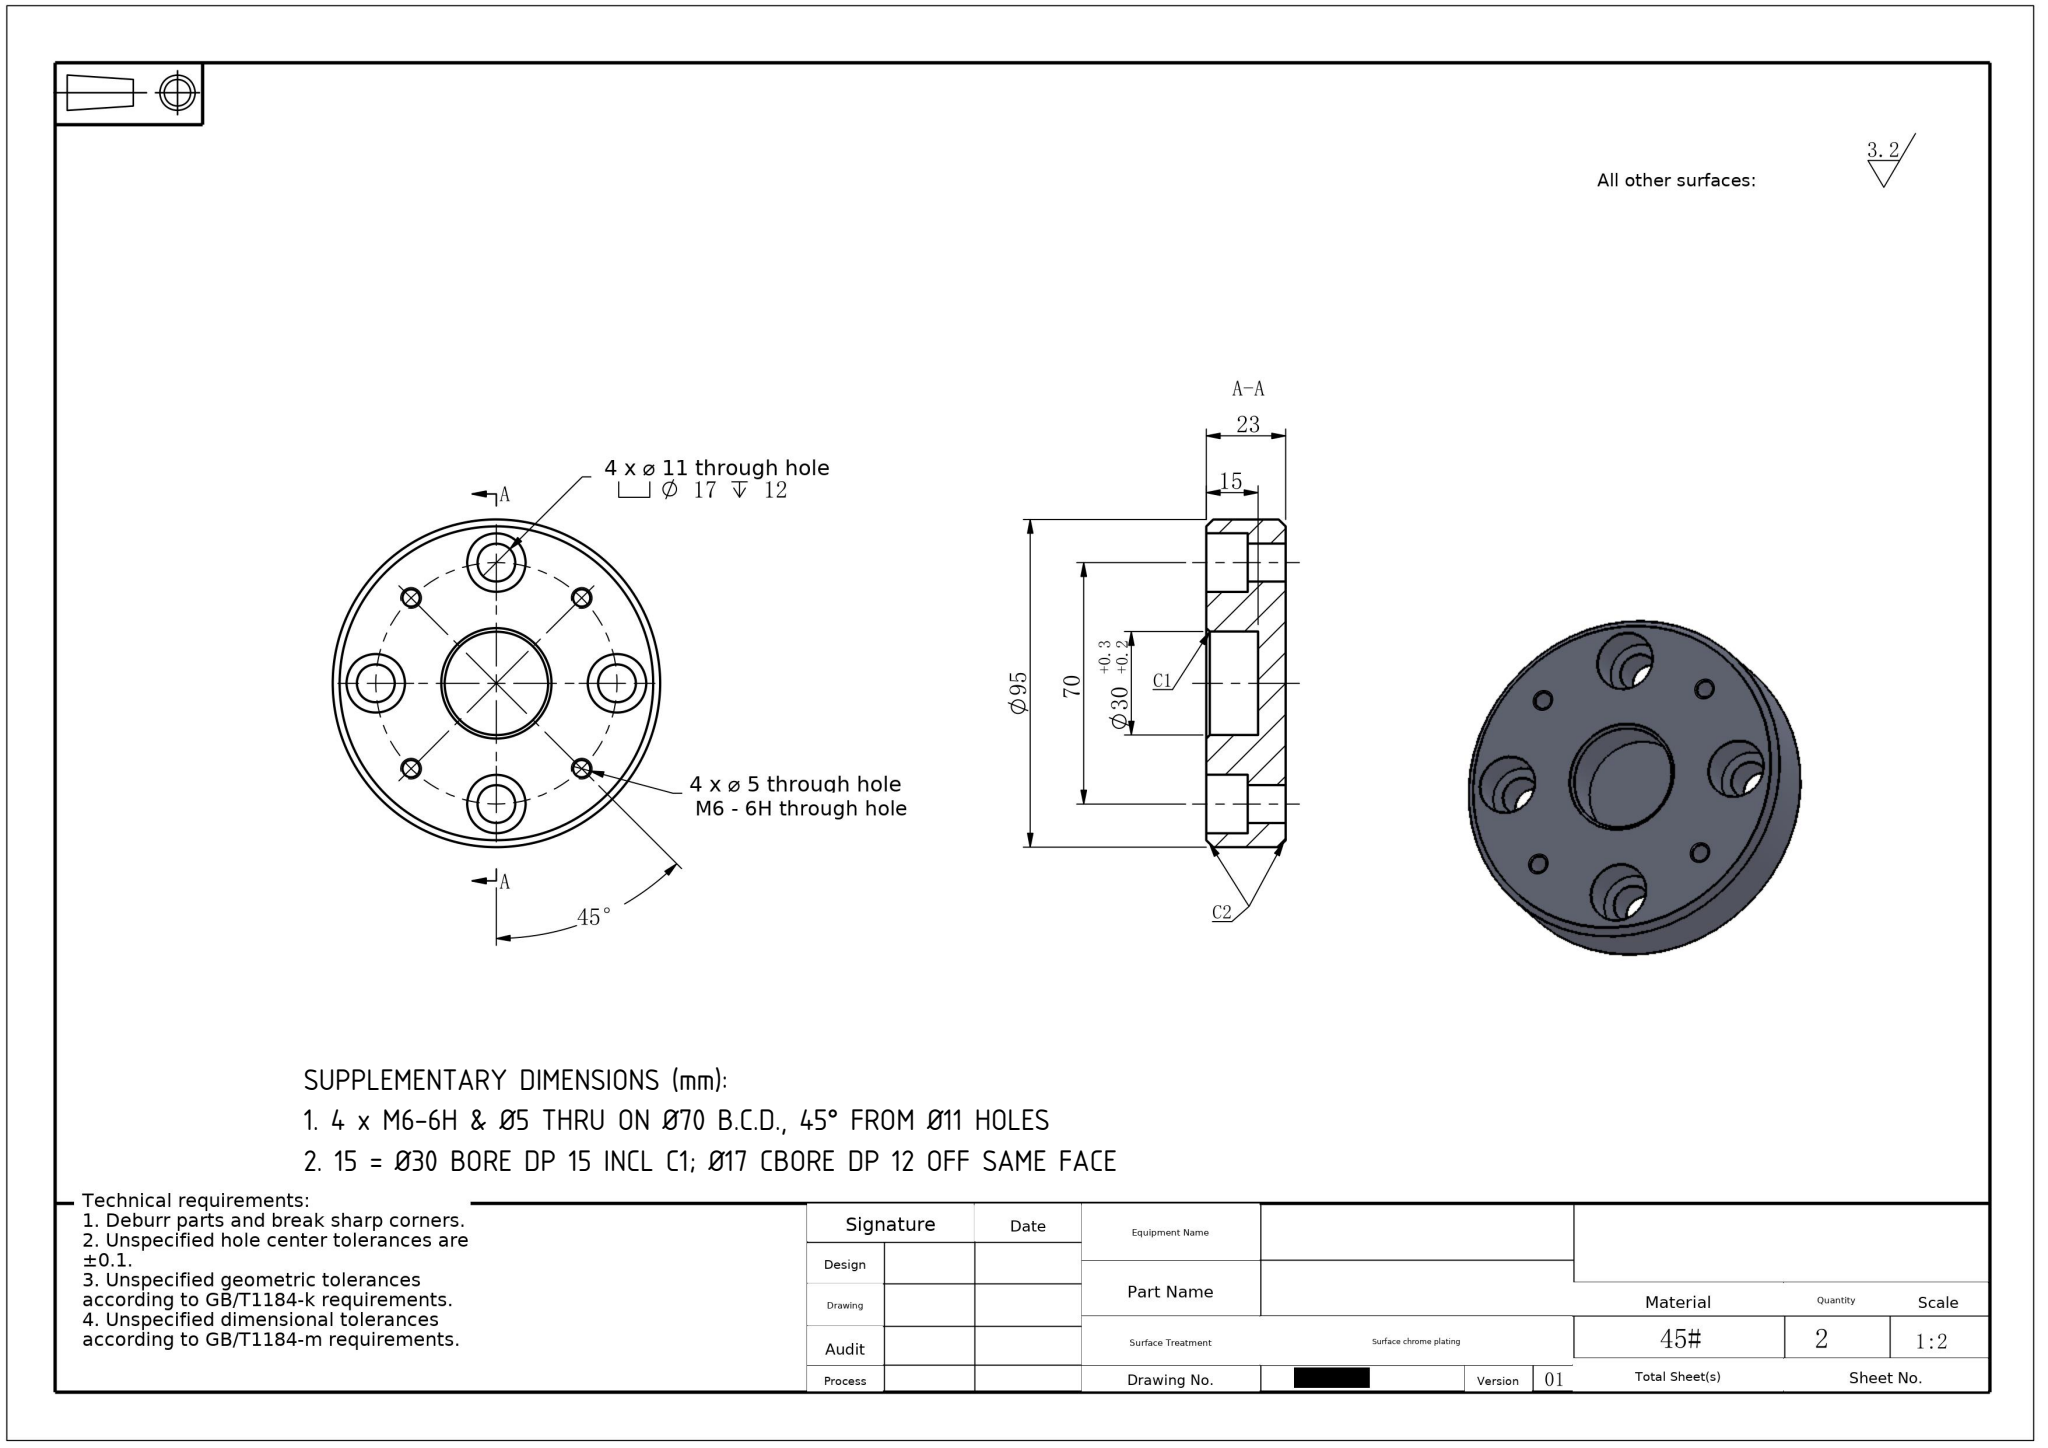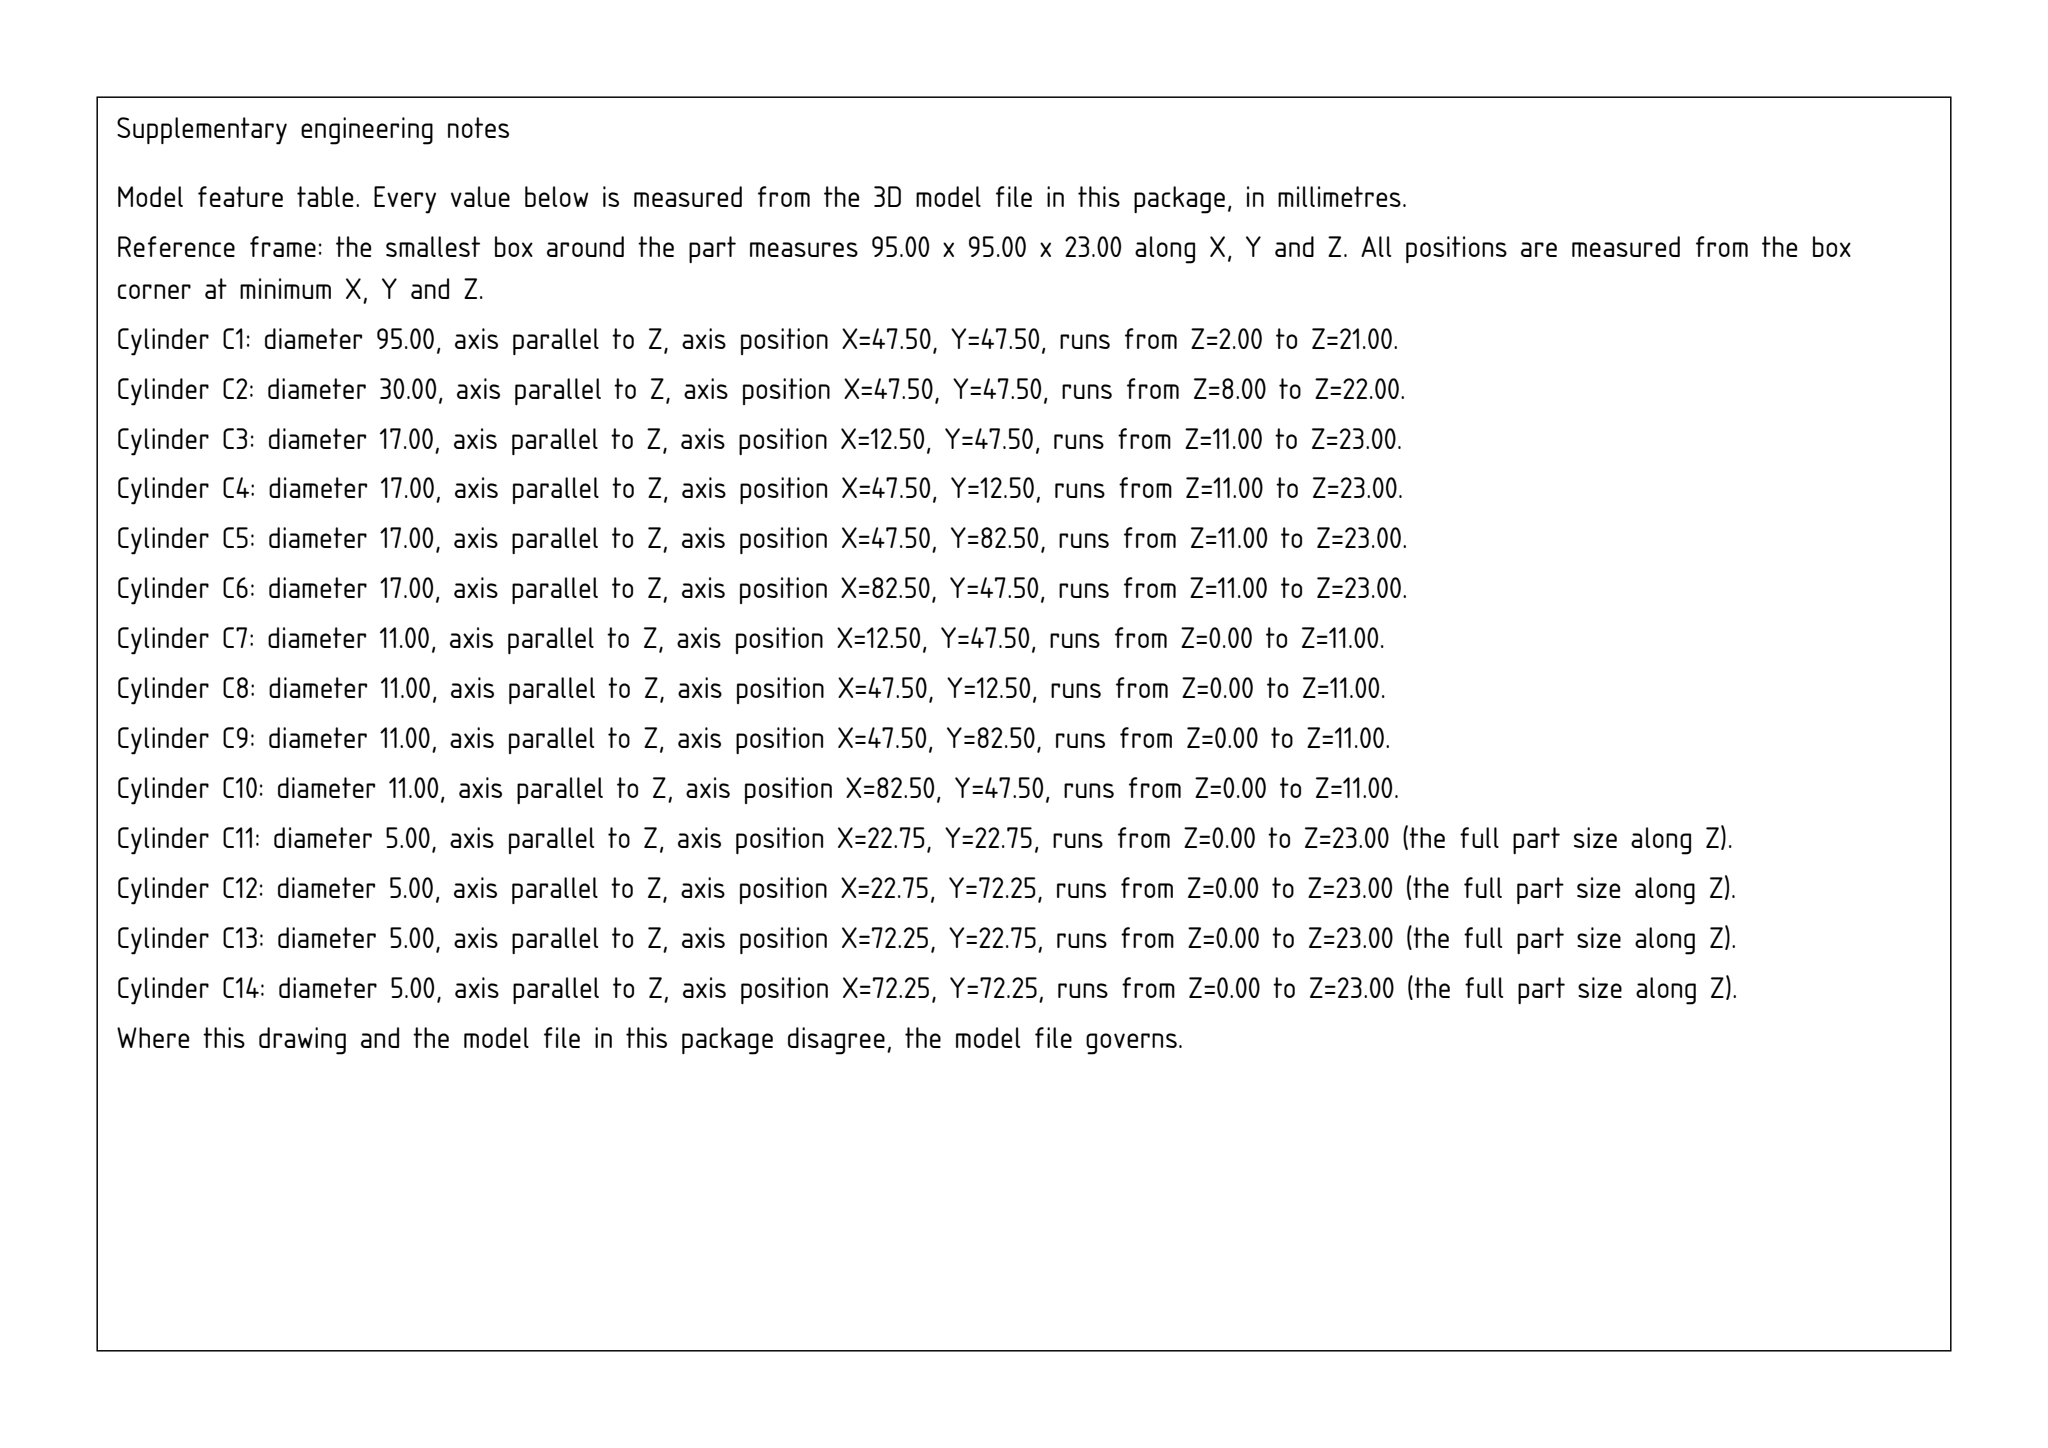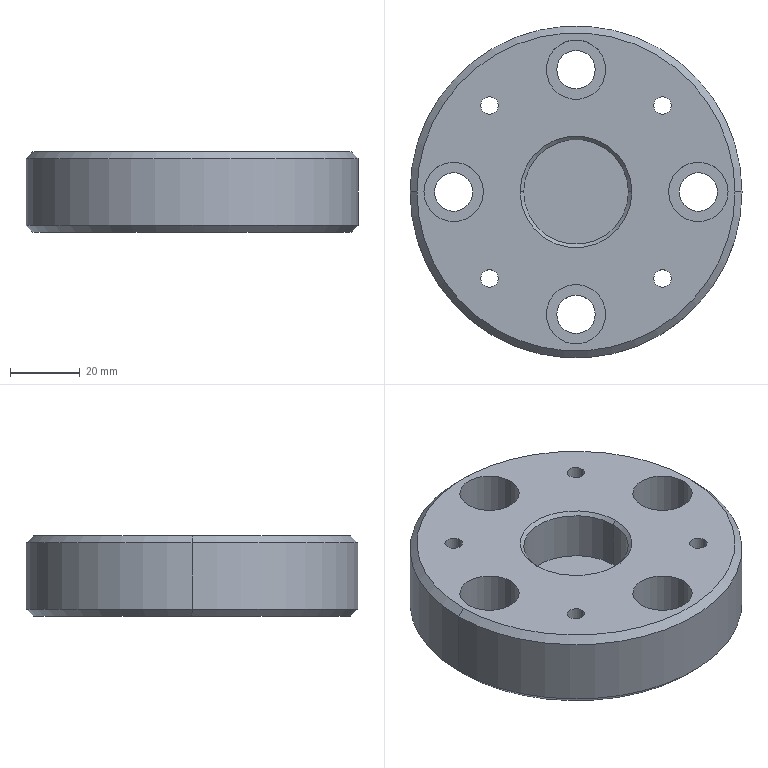Part | SolidWorks | mm | 1 solid | 41 faces | box 95 x 95 x 23 mm | volume 134318 mm3 | cylinder 28 | plane 7 | cone 6 | commonest cylinder face diameters 5 x8 17 x8 11 x8 30 x2 95 x2
build123d program:
from build123d import *

# Parameters (mm, degrees)
SKETCH1_R                                        = 47.5
BOSS_EXTRUDE1_DEPTH                              = 23
SKETCH2_R                                        = 15
CUT_EXTRUDE1_DEPTH                               = 15
CHAMFER1_SIZE                                    = 1
M10_HEX_SOCKET_HEAD_CAP_SCREW_CBORE1_D           = 11
M10_HEX_SOCKET_HEAD_CAP_SCREW_CBORE1_CBORE_D     = 17
M10_HEX_SOCKET_HEAD_CAP_SCREW_CBORE1_CBORE_DEPTH = 12
CIRPATTERN1_COUNT                                = 4
M6_TAPPED_HOLE1_D                                = 5
CIRPATTERN2_COUNT                                = 4
CHAMFER2_SIZE                                    = 2


with BuildPart() as part:
    # Sketch1 → Boss-Extrude1 (new body)
    with BuildSketch(Plane.XY):
        Circle(SKETCH1_R)
    extrude(amount=BOSS_EXTRUDE1_DEPTH)

    # Sketch2 → Cut-Extrude1 (cut)
    with BuildSketch(Plane.XY.offset(23)):
        Circle(SKETCH2_R)
    extrude(amount=-CUT_EXTRUDE1_DEPTH, mode=Mode.SUBTRACT)

    # Chamfer1
    chamfer1_edges = [part.edges().sort_by_distance(p)[0] for p in [
        (-15, 0, 23),
    ]]
    chamfer(chamfer1_edges, length=CHAMFER1_SIZE)

    # M10 Hex Socket Head Cap Screw CBORE1 (through all)
    with Locations(Plane.XY.offset(23)):
        with Locations((0, 35)):
            m10_hex_socket_head_cap_screw_cbore1 = CounterBoreHole(M10_HEX_SOCKET_HEAD_CAP_SCREW_CBORE1_D / 2, M10_HEX_SOCKET_HEAD_CAP_SCREW_CBORE1_CBORE_D / 2, M10_HEX_SOCKET_HEAD_CAP_SCREW_CBORE1_CBORE_DEPTH)

    # CirPattern1: M10 Hex Socket Head Cap Screw CBORE1 ×4 about axis
    cirpattern1_axis = Axis((0, 0, 0), (0, 0, 1))
    for i in range(1, CIRPATTERN1_COUNT):
        add(m10_hex_socket_head_cap_screw_cbore1.rotate(cirpattern1_axis, i * 360 / CIRPATTERN1_COUNT), mode=Mode.SUBTRACT)

    # M6 Tapped Hole1 (through all)
    with Locations(Plane.XY.offset(23)):
        with Locations((-24.749, -24.749)):
            m6_tapped_hole1 = Hole(M6_TAPPED_HOLE1_D / 2)

    # CirPattern2: M6 Tapped Hole1 ×4 about axis
    cirpattern2_axis = Axis((0, 0, 0), (0, 0, 1))
    for i in range(1, CIRPATTERN2_COUNT):
        add(m6_tapped_hole1.rotate(cirpattern2_axis, i * 360 / CIRPATTERN2_COUNT), mode=Mode.SUBTRACT)

    # Chamfer2
    chamfer2_edges = [part.edges().sort_by_distance(p)[0] for p in [
        (-47.5, 0, 0),
        (-47.5, 0, 23),
    ]]
    chamfer(chamfer2_edges, length=CHAMFER2_SIZE)


solid = part.part